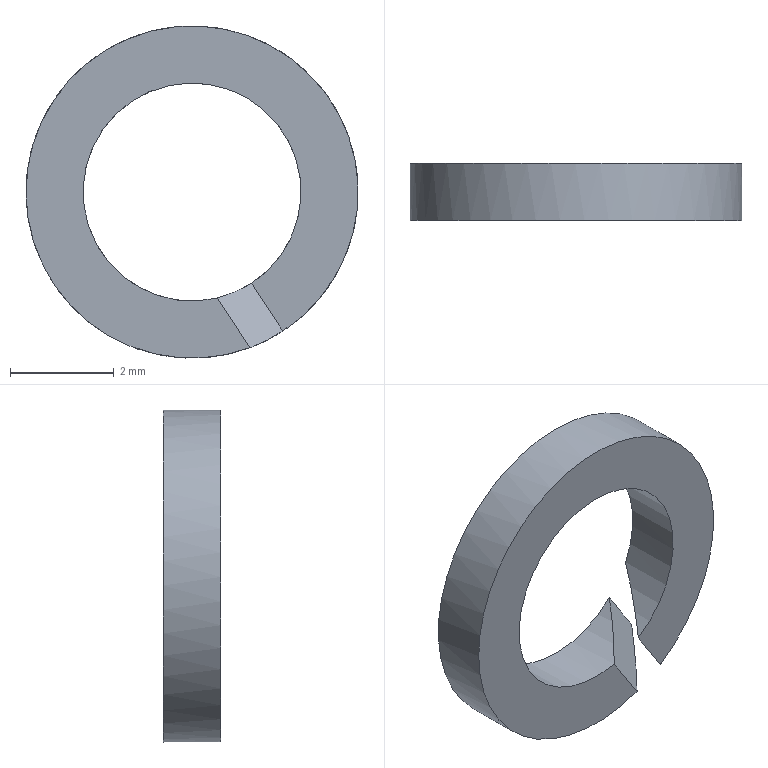Component | NX | SPRING_WASHER_4 | 1 solid | 6 faces | box 6.4 x 1.1 x 6.4 mm | volume 19 mm3 | plane 4 | cylinder 2 | commonest cylinder face diameters 6.4 x1 4.2 x1
STEP:
#1=CARTESIAN_POINT('',(0.,0.,0.));
#2=DIRECTION('',(0.,0.,1.));
#3=DIRECTION('',(1.,0.,0.));
#4=AXIS2_PLACEMENT_3D('',#1,#2,#3);
#5=CARTESIAN_POINT('',(21.566,-66.923,-95.444));
#6=VERTEX_POINT('',#5);
#7=CARTESIAN_POINT('',(22.064,-66.923,-94.914));
#8=VERTEX_POINT('',#7);
#9=CARTESIAN_POINT('',(19.5,-66.923,-93.));
#10=DIRECTION('',(0.,1.,0.));
#11=DIRECTION('',(0.5469,0.,-0.8372));
#12=AXIS2_PLACEMENT_3D('',#9,#10,#11);
#13=CIRCLE('',#12,3.2);
#14=CARTESIAN_POINT('',(19.5,-66.923,-93.));
#15=DIRECTION('',(0.,-1.,0.));
#16=DIRECTION('',(0.5469,0.,-0.8372));
#17=AXIS2_PLACEMENT_3D('',#14,#15,#16);
#18=CYLINDRICAL_SURFACE('',#17,3.2);
#19=CARTESIAN_POINT('',(12.566,0.));
#20=DIRECTION('',(-1.,0.));
#21=VECTOR('',#20,1.);
#22=LINE('',#19,#21);
#23=(GEOMETRIC_REPRESENTATION_CONTEXT(2)PARAMETRIC_REPRESENTATION_CONTEXT()REPRESENTATION_CONTEXT('',''));
#24=DEFINITIONAL_REPRESENTATION('',(#22),#23);
#25=PCURVE('',#18,#24);
#26=CARTESIAN_POINT('',(19.5,-66.923,-93.));
#27=DIRECTION('',(0.,-1.,0.));
#28=DIRECTION('',(0.5469,0.,-0.8372));
#29=AXIS2_PLACEMENT_3D('',#26,#27,#28);
#30=PLANE('',#29);
#31=CARTESIAN_POINT('',(3.2,-0.));
#32=CARTESIAN_POINT('',(3.2,-5.543));
#33=CARTESIAN_POINT('',(-1.6,-2.771));
#34=CARTESIAN_POINT('',(-6.4,0.));
#35=CARTESIAN_POINT('',(-1.6,2.771));
#36=CARTESIAN_POINT('',(3.2,5.543));
#37=CARTESIAN_POINT('',(3.2,-0.));
#38=(BOUNDED_CURVE()B_SPLINE_CURVE(2,(#31,#32,#33,#34,#35,#36,#37),.UNSPECIFIED.,.T.,.F.)B_SPLINE_CURVE_WITH_KNOTS((1,2,2,2,2,1),(-2.094,0.,2.094,4.189,6.283,8.378),.UNSPECIFIED.)CURVE()GEOMETRIC_REPRESENTATION_ITEM()RATIONAL_B_SPLINE_CURVE((1.,0.5,1.,0.5,1.,0.5,1.))REPRESENTATION_ITEM(''));
#39=(GEOMETRIC_REPRESENTATION_CONTEXT(2)PARAMETRIC_REPRESENTATION_CONTEXT()REPRESENTATION_CONTEXT('',''));
#40=DEFINITIONAL_REPRESENTATION('',(#38),#39);
#41=PCURVE('',#30,#40);
#42=SURFACE_CURVE('',#13,(#25,#41),.PCURVE_S1.);
#43=EDGE_CURVE('',#6,#8,#42,.T.);
#44=ORIENTED_EDGE('',*,*,#43,.F.);
#45=CARTESIAN_POINT('',(20.615,-68.023,-95.999));
#46=VERTEX_POINT('',#45);
#47=CARTESIAN_POINT('',(19.5,-67.316,-93.));
#48=DIRECTION('',(0.592,-0.7071,0.3867));
#49=DIRECTION('',(-0.592,-0.7071,-0.3867));
#50=AXIS2_PLACEMENT_3D('',#47,#48,#49);
#51=ELLIPSE('',#50,4.525,3.2);
#52=CARTESIAN_POINT('',(6.06,1.1));
#53=CARTESIAN_POINT('',(6.406,-0.));
#54=B_SPLINE_CURVE_WITH_KNOTS('',1,(#52,#53),.UNSPECIFIED.,.F.,.F.,(2,2),(1.348,1.694),.PIECEWISE_BEZIER_KNOTS.);
#55=(GEOMETRIC_REPRESENTATION_CONTEXT(2)PARAMETRIC_REPRESENTATION_CONTEXT()REPRESENTATION_CONTEXT('',''));
#56=DEFINITIONAL_REPRESENTATION('',(#54),#55);
#57=PCURVE('',#18,#56);
#58=CARTESIAN_POINT('',(23.341,-68.804,-101.6));
#59=DIRECTION('',(0.592,-0.7071,0.3867));
#60=DIRECTION('',(-0.592,-0.7071,-0.3867));
#61=AXIS2_PLACEMENT_3D('',#58,#59,#60);
#62=PLANE('',#61);
#63=CARTESIAN_POINT('',(-2.105,-9.3));
#64=DIRECTION('',(1.,-0.));
#65=AXIS2_PLACEMENT_2D('',#63,#64);
#66=ELLIPSE('',#65,4.525,3.2);
#67=(GEOMETRIC_REPRESENTATION_CONTEXT(2)PARAMETRIC_REPRESENTATION_CONTEXT()REPRESENTATION_CONTEXT('',''));
#68=DEFINITIONAL_REPRESENTATION('',(#66),#67);
#69=PCURVE('',#62,#68);
#70=SURFACE_CURVE('',#51,(#57,#69),.PCURVE_S1.);
#71=EDGE_CURVE('',#46,#6,#70,.T.);
#72=ORIENTED_EDGE('',*,*,#71,.F.);
#73=CARTESIAN_POINT('',(21.25,-68.023,-95.679));
#74=VERTEX_POINT('',#73);
#75=CARTESIAN_POINT('',(19.5,-68.023,-93.));
#76=DIRECTION('',(0.,1.,0.));
#77=DIRECTION('',(0.5469,0.,-0.8372));
#78=AXIS2_PLACEMENT_3D('',#75,#76,#77);
#79=CIRCLE('',#78,3.2);
#80=CARTESIAN_POINT('',(6.283,1.1));
#81=DIRECTION('',(-1.,0.));
#82=VECTOR('',#81,1.);
#83=LINE('',#80,#82);
#84=(GEOMETRIC_REPRESENTATION_CONTEXT(2)PARAMETRIC_REPRESENTATION_CONTEXT()REPRESENTATION_CONTEXT('',''));
#85=DEFINITIONAL_REPRESENTATION('',(#83),#84);
#86=PCURVE('',#18,#85);
#87=CARTESIAN_POINT('',(19.5,-68.023,-93.));
#88=DIRECTION('',(0.,-1.,0.));
#89=DIRECTION('',(0.5469,0.,-0.8372));
#90=AXIS2_PLACEMENT_3D('',#87,#88,#89);
#91=PLANE('',#90);
#92=CARTESIAN_POINT('',(3.2,-0.));
#93=CARTESIAN_POINT('',(3.2,-5.543));
#94=CARTESIAN_POINT('',(-1.6,-2.771));
#95=CARTESIAN_POINT('',(-6.4,0.));
#96=CARTESIAN_POINT('',(-1.6,2.771));
#97=CARTESIAN_POINT('',(3.2,5.543));
#98=CARTESIAN_POINT('',(3.2,-0.));
#99=(BOUNDED_CURVE()B_SPLINE_CURVE(2,(#92,#93,#94,#95,#96,#97,#98),.UNSPECIFIED.,.T.,.F.)B_SPLINE_CURVE_WITH_KNOTS((1,2,2,2,2,1),(-2.094,0.,2.094,4.189,6.283,8.378),.UNSPECIFIED.)CURVE()GEOMETRIC_REPRESENTATION_ITEM()RATIONAL_B_SPLINE_CURVE((1.,0.5,1.,0.5,1.,0.5,1.))REPRESENTATION_ITEM(''));
#100=(GEOMETRIC_REPRESENTATION_CONTEXT(2)PARAMETRIC_REPRESENTATION_CONTEXT()REPRESENTATION_CONTEXT('',''));
#101=DEFINITIONAL_REPRESENTATION('',(#99),#100);
#102=PCURVE('',#91,#101);
#103=SURFACE_CURVE('',#79,(#86,#102),.PCURVE_S1.);
#104=EDGE_CURVE('',#46,#74,#103,.T.);
#105=ORIENTED_EDGE('',*,*,#104,.T.);
#106=CARTESIAN_POINT('',(19.5,-68.023,-93.));
#107=DIRECTION('',(-0.592,0.7071,-0.3867));
#108=DIRECTION('',(-0.592,-0.7071,-0.3867));
#109=AXIS2_PLACEMENT_3D('',#106,#107,#108);
#110=ELLIPSE('',#109,4.525,3.2);
#111=CARTESIAN_POINT('',(0.3509,-0.));
#112=CARTESIAN_POINT('',(0.,1.1));
#113=B_SPLINE_CURVE_WITH_KNOTS('',1,(#111,#112),.UNSPECIFIED.,.F.,.F.,(2,2),(4.361,4.712),.PIECEWISE_BEZIER_KNOTS.);
#114=(GEOMETRIC_REPRESENTATION_CONTEXT(2)PARAMETRIC_REPRESENTATION_CONTEXT()REPRESENTATION_CONTEXT('',''));
#115=DEFINITIONAL_REPRESENTATION('',(#113),#114);
#116=PCURVE('',#18,#115);
#117=CARTESIAN_POINT('',(26.917,-65.239,-99.263));
#118=DIRECTION('',(-0.592,0.7071,-0.3867));
#119=DIRECTION('',(0.592,0.7071,0.3867));
#120=AXIS2_PLACEMENT_3D('',#117,#118,#119);
#121=PLANE('',#120);
#122=CARTESIAN_POINT('',(-3.936,-9.3));
#123=DIRECTION('',(-1.,-0.));
#124=AXIS2_PLACEMENT_2D('',#122,#123);
#125=ELLIPSE('',#124,4.525,3.2);
#126=(GEOMETRIC_REPRESENTATION_CONTEXT(2)PARAMETRIC_REPRESENTATION_CONTEXT()REPRESENTATION_CONTEXT('',''));
#127=DEFINITIONAL_REPRESENTATION('',(#125),#126);
#128=PCURVE('',#121,#127);
#129=SURFACE_CURVE('',#110,(#116,#128),.PCURVE_S1.);
#130=EDGE_CURVE('',#8,#74,#129,.T.);
#131=ORIENTED_EDGE('',*,*,#130,.F.);
#132=EDGE_LOOP('',(#44,#72,#105,#131));
#133=FACE_BOUND('',#132,.T.);
#134=ADVANCED_FACE('',(#133),#18,.T.);
#135=CARTESIAN_POINT('',(19.99,-68.023,-95.042));
#136=VERTEX_POINT('',#135);
#137=CARTESIAN_POINT('',(20.649,-68.023,-94.758));
#138=VERTEX_POINT('',#137);
#139=CARTESIAN_POINT('',(19.5,-68.023,-93.));
#140=DIRECTION('',(0.,1.,0.));
#141=DIRECTION('',(0.5469,0.,-0.8372));
#142=AXIS2_PLACEMENT_3D('',#139,#140,#141);
#143=CIRCLE('',#142,2.1);
#144=CARTESIAN_POINT('',(19.5,-66.923,-93.));
#145=DIRECTION('',(0.,-1.,0.));
#146=DIRECTION('',(0.5469,0.,-0.8372));
#147=AXIS2_PLACEMENT_3D('',#144,#145,#146);
#148=CYLINDRICAL_SURFACE('',#147,2.1);
#149=CARTESIAN_POINT('',(6.283,1.1));
#150=DIRECTION('',(-1.,0.));
#151=VECTOR('',#150,1.);
#152=LINE('',#149,#151);
#153=(GEOMETRIC_REPRESENTATION_CONTEXT(2)PARAMETRIC_REPRESENTATION_CONTEXT()REPRESENTATION_CONTEXT('',''));
#154=DEFINITIONAL_REPRESENTATION('',(#152),#153);
#155=PCURVE('',#148,#154);
#156=CARTESIAN_POINT('',(2.1,-0.));
#157=CARTESIAN_POINT('',(2.1,-3.637));
#158=CARTESIAN_POINT('',(-1.05,-1.819));
#159=CARTESIAN_POINT('',(-4.2,0.));
#160=CARTESIAN_POINT('',(-1.05,1.819));
#161=CARTESIAN_POINT('',(2.1,3.637));
#162=CARTESIAN_POINT('',(2.1,-0.));
#163=(BOUNDED_CURVE()B_SPLINE_CURVE(2,(#156,#157,#158,#159,#160,#161,#162),.UNSPECIFIED.,.T.,.F.)B_SPLINE_CURVE_WITH_KNOTS((1,2,2,2,2,1),(-2.094,0.,2.094,4.189,6.283,8.378),.UNSPECIFIED.)CURVE()GEOMETRIC_REPRESENTATION_ITEM()RATIONAL_B_SPLINE_CURVE((1.,0.5,1.,0.5,1.,0.5,1.))REPRESENTATION_ITEM(''));
#164=(GEOMETRIC_REPRESENTATION_CONTEXT(2)PARAMETRIC_REPRESENTATION_CONTEXT()REPRESENTATION_CONTEXT('',''));
#165=DEFINITIONAL_REPRESENTATION('',(#163),#164);
#166=PCURVE('',#91,#165);
#167=SURFACE_CURVE('',#143,(#155,#166),.PCURVE_S1.);
#168=EDGE_CURVE('',#136,#138,#167,.T.);
#169=ORIENTED_EDGE('',*,*,#168,.T.);
#170=CARTESIAN_POINT('',(21.399,-66.923,-93.896));
#171=VERTEX_POINT('',#170);
#172=CARTESIAN_POINT('',(19.5,-68.023,-93.));
#173=DIRECTION('',(-0.592,0.7071,-0.3867));
#174=DIRECTION('',(-0.592,-0.7071,-0.3867));
#175=AXIS2_PLACEMENT_3D('',#172,#173,#174);
#176=ELLIPSE('',#175,2.97,2.1);
#177=CARTESIAN_POINT('',(0.5513,0.));
#178=CARTESIAN_POINT('',(0.,1.1));
#179=B_SPLINE_CURVE_WITH_KNOTS('',1,(#177,#178),.UNSPECIFIED.,.F.,.F.,(2,2),(4.161,4.712),.PIECEWISE_BEZIER_KNOTS.);
#180=(GEOMETRIC_REPRESENTATION_CONTEXT(2)PARAMETRIC_REPRESENTATION_CONTEXT()REPRESENTATION_CONTEXT('',''));
#181=DEFINITIONAL_REPRESENTATION('',(#179),#180);
#182=PCURVE('',#148,#181);
#183=CARTESIAN_POINT('',(-3.936,-9.3));
#184=DIRECTION('',(-1.,-0.));
#185=AXIS2_PLACEMENT_2D('',#183,#184);
#186=ELLIPSE('',#185,2.97,2.1);
#187=(GEOMETRIC_REPRESENTATION_CONTEXT(2)PARAMETRIC_REPRESENTATION_CONTEXT()REPRESENTATION_CONTEXT('',''));
#188=DEFINITIONAL_REPRESENTATION('',(#186),#187);
#189=PCURVE('',#121,#188);
#190=SURFACE_CURVE('',#176,(#182,#189),.PCURVE_S1.);
#191=EDGE_CURVE('',#171,#138,#190,.T.);
#192=ORIENTED_EDGE('',*,*,#191,.F.);
#193=CARTESIAN_POINT('',(20.957,-66.923,-94.512));
#194=VERTEX_POINT('',#193);
#195=CARTESIAN_POINT('',(19.5,-66.923,-93.));
#196=DIRECTION('',(0.,1.,0.));
#197=DIRECTION('',(0.5469,0.,-0.8372));
#198=AXIS2_PLACEMENT_3D('',#195,#196,#197);
#199=CIRCLE('',#198,2.1);
#200=CARTESIAN_POINT('',(12.566,0.));
#201=DIRECTION('',(-1.,0.));
#202=VECTOR('',#201,1.);
#203=LINE('',#200,#202);
#204=(GEOMETRIC_REPRESENTATION_CONTEXT(2)PARAMETRIC_REPRESENTATION_CONTEXT()REPRESENTATION_CONTEXT('',''));
#205=DEFINITIONAL_REPRESENTATION('',(#203),#204);
#206=PCURVE('',#148,#205);
#207=CARTESIAN_POINT('',(2.1,-0.));
#208=CARTESIAN_POINT('',(2.1,-3.637));
#209=CARTESIAN_POINT('',(-1.05,-1.819));
#210=CARTESIAN_POINT('',(-4.2,0.));
#211=CARTESIAN_POINT('',(-1.05,1.819));
#212=CARTESIAN_POINT('',(2.1,3.637));
#213=CARTESIAN_POINT('',(2.1,-0.));
#214=(BOUNDED_CURVE()B_SPLINE_CURVE(2,(#207,#208,#209,#210,#211,#212,#213),.UNSPECIFIED.,.T.,.F.)B_SPLINE_CURVE_WITH_KNOTS((1,2,2,2,2,1),(-2.094,0.,2.094,4.189,6.283,8.378),.UNSPECIFIED.)CURVE()GEOMETRIC_REPRESENTATION_ITEM()RATIONAL_B_SPLINE_CURVE((1.,0.5,1.,0.5,1.,0.5,1.))REPRESENTATION_ITEM(''));
#215=(GEOMETRIC_REPRESENTATION_CONTEXT(2)PARAMETRIC_REPRESENTATION_CONTEXT()REPRESENTATION_CONTEXT('',''));
#216=DEFINITIONAL_REPRESENTATION('',(#214),#215);
#217=PCURVE('',#30,#216);
#218=SURFACE_CURVE('',#199,(#206,#217),.PCURVE_S1.);
#219=EDGE_CURVE('',#194,#171,#218,.T.);
#220=ORIENTED_EDGE('',*,*,#219,.F.);
#221=CARTESIAN_POINT('',(19.5,-67.316,-93.));
#222=DIRECTION('',(0.592,-0.7071,0.3867));
#223=DIRECTION('',(-0.592,-0.7071,-0.3867));
#224=AXIS2_PLACEMENT_3D('',#221,#222,#223);
#225=ELLIPSE('',#224,2.97,2.1);
#226=CARTESIAN_POINT('',(5.94,1.1));
#227=CARTESIAN_POINT('',(6.471,-0.));
#228=B_SPLINE_CURVE_WITH_KNOTS('',1,(#226,#227),.UNSPECIFIED.,.F.,.F.,(2,2),(1.227,1.759),.PIECEWISE_BEZIER_KNOTS.);
#229=(GEOMETRIC_REPRESENTATION_CONTEXT(2)PARAMETRIC_REPRESENTATION_CONTEXT()REPRESENTATION_CONTEXT('',''));
#230=DEFINITIONAL_REPRESENTATION('',(#228),#229);
#231=PCURVE('',#148,#230);
#232=CARTESIAN_POINT('',(-2.105,-9.3));
#233=DIRECTION('',(1.,-0.));
#234=AXIS2_PLACEMENT_2D('',#232,#233);
#235=ELLIPSE('',#234,2.97,2.1);
#236=(GEOMETRIC_REPRESENTATION_CONTEXT(2)PARAMETRIC_REPRESENTATION_CONTEXT()REPRESENTATION_CONTEXT('',''));
#237=DEFINITIONAL_REPRESENTATION('',(#235),#236);
#238=PCURVE('',#62,#237);
#239=SURFACE_CURVE('',#225,(#231,#238),.PCURVE_S1.);
#240=EDGE_CURVE('',#136,#194,#239,.T.);
#241=ORIENTED_EDGE('',*,*,#240,.F.);
#242=EDGE_LOOP('',(#169,#192,#220,#241));
#243=FACE_BOUND('',#242,.F.);
#244=ADVANCED_FACE('',(#243),#148,.F.);
#245=CARTESIAN_POINT('',(19.829,-66.923,-92.785));
#246=DIRECTION('',(-0.5469,0.,0.8372));
#247=VECTOR('',#246,1.);
#248=LINE('',#245,#247);
#249=CARTESIAN_POINT('',(-0.,0.3929));
#250=DIRECTION('',(-1.,0.));
#251=VECTOR('',#250,1.);
#252=LINE('',#249,#251);
#253=(GEOMETRIC_REPRESENTATION_CONTEXT(2)PARAMETRIC_REPRESENTATION_CONTEXT()REPRESENTATION_CONTEXT('',''));
#254=DEFINITIONAL_REPRESENTATION('',(#252),#253);
#255=PCURVE('',#30,#254);
#256=CARTESIAN_POINT('',(-2.66,-9.3));
#257=DIRECTION('',(0.,-1.));
#258=VECTOR('',#257,1.);
#259=LINE('',#256,#258);
#260=(GEOMETRIC_REPRESENTATION_CONTEXT(2)PARAMETRIC_REPRESENTATION_CONTEXT()REPRESENTATION_CONTEXT('',''));
#261=DEFINITIONAL_REPRESENTATION('',(#259),#260);
#262=PCURVE('',#62,#261);
#263=SURFACE_CURVE('',#248,(#255,#262),.PCURVE_S1.);
#264=EDGE_CURVE('',#6,#194,#263,.T.);
#265=ORIENTED_EDGE('',*,*,#264,.F.);
#266=ORIENTED_EDGE('',*,*,#43,.T.);
#267=CARTESIAN_POINT('',(20.421,-66.923,-92.398));
#268=DIRECTION('',(0.5469,0.,-0.8372));
#269=VECTOR('',#268,1.);
#270=LINE('',#267,#269);
#271=CARTESIAN_POINT('',(0.,1.1));
#272=DIRECTION('',(1.,0.));
#273=VECTOR('',#272,1.);
#274=LINE('',#271,#273);
#275=(GEOMETRIC_REPRESENTATION_CONTEXT(2)PARAMETRIC_REPRESENTATION_CONTEXT()REPRESENTATION_CONTEXT('',''));
#276=DEFINITIONAL_REPRESENTATION('',(#274),#275);
#277=PCURVE('',#30,#276);
#278=CARTESIAN_POINT('',(-2.38,-9.3));
#279=DIRECTION('',(0.,1.));
#280=VECTOR('',#279,1.);
#281=LINE('',#278,#280);
#282=(GEOMETRIC_REPRESENTATION_CONTEXT(2)PARAMETRIC_REPRESENTATION_CONTEXT()REPRESENTATION_CONTEXT('',''));
#283=DEFINITIONAL_REPRESENTATION('',(#281),#282);
#284=PCURVE('',#121,#283);
#285=SURFACE_CURVE('',#270,(#277,#284),.PCURVE_S1.);
#286=EDGE_CURVE('',#171,#8,#285,.T.);
#287=ORIENTED_EDGE('',*,*,#286,.F.);
#288=ORIENTED_EDGE('',*,*,#219,.F.);
#289=EDGE_LOOP('',(#265,#266,#287,#288));
#290=FACE_BOUND('',#289,.T.);
#291=ADVANCED_FACE('',(#290),#30,.F.);
#292=ORIENTED_EDGE('',*,*,#104,.F.);
#293=CARTESIAN_POINT('',(18.908,-68.023,-93.387));
#294=DIRECTION('',(-0.5469,0.,0.8372));
#295=VECTOR('',#294,1.);
#296=LINE('',#293,#295);
#297=CARTESIAN_POINT('',(0.,-0.7071));
#298=DIRECTION('',(-1.,0.));
#299=VECTOR('',#298,1.);
#300=LINE('',#297,#299);
#301=(GEOMETRIC_REPRESENTATION_CONTEXT(2)PARAMETRIC_REPRESENTATION_CONTEXT()REPRESENTATION_CONTEXT('',''));
#302=DEFINITIONAL_REPRESENTATION('',(#300),#301);
#303=PCURVE('',#91,#302);
#304=CARTESIAN_POINT('',(-1.105,-9.3));
#305=DIRECTION('',(0.,-1.));
#306=VECTOR('',#305,1.);
#307=LINE('',#304,#306);
#308=(GEOMETRIC_REPRESENTATION_CONTEXT(2)PARAMETRIC_REPRESENTATION_CONTEXT()REPRESENTATION_CONTEXT('',''));
#309=DEFINITIONAL_REPRESENTATION('',(#307),#308);
#310=PCURVE('',#62,#309);
#311=SURFACE_CURVE('',#296,(#303,#310),.PCURVE_S1.);
#312=EDGE_CURVE('',#46,#136,#311,.T.);
#313=ORIENTED_EDGE('',*,*,#312,.T.);
#314=ORIENTED_EDGE('',*,*,#168,.T.);
#315=CARTESIAN_POINT('',(19.5,-68.023,-93.));
#316=DIRECTION('',(0.5469,0.,-0.8372));
#317=VECTOR('',#316,1.);
#318=LINE('',#315,#317);
#319=CARTESIAN_POINT('',(0.,0.));
#320=DIRECTION('',(1.,0.));
#321=VECTOR('',#320,1.);
#322=LINE('',#319,#321);
#323=(GEOMETRIC_REPRESENTATION_CONTEXT(2)PARAMETRIC_REPRESENTATION_CONTEXT()REPRESENTATION_CONTEXT('',''));
#324=DEFINITIONAL_REPRESENTATION('',(#322),#323);
#325=PCURVE('',#91,#324);
#326=CARTESIAN_POINT('',(-3.936,-9.3));
#327=DIRECTION('',(0.,1.));
#328=VECTOR('',#327,1.);
#329=LINE('',#326,#328);
#330=(GEOMETRIC_REPRESENTATION_CONTEXT(2)PARAMETRIC_REPRESENTATION_CONTEXT()REPRESENTATION_CONTEXT('',''));
#331=DEFINITIONAL_REPRESENTATION('',(#329),#330);
#332=PCURVE('',#121,#331);
#333=SURFACE_CURVE('',#318,(#325,#332),.PCURVE_S1.);
#334=EDGE_CURVE('',#138,#74,#333,.T.);
#335=ORIENTED_EDGE('',*,*,#334,.T.);
#336=EDGE_LOOP('',(#292,#313,#314,#335));
#337=FACE_BOUND('',#336,.T.);
#338=ADVANCED_FACE('',(#337),#91,.T.);
#339=ORIENTED_EDGE('',*,*,#286,.T.);
#340=ORIENTED_EDGE('',*,*,#130,.T.);
#341=ORIENTED_EDGE('',*,*,#334,.F.);
#342=ORIENTED_EDGE('',*,*,#191,.F.);
#343=EDGE_LOOP('',(#339,#340,#341,#342));
#344=FACE_BOUND('',#343,.T.);
#345=ADVANCED_FACE('',(#344),#121,.T.);
#346=ORIENTED_EDGE('',*,*,#264,.T.);
#347=ORIENTED_EDGE('',*,*,#240,.F.);
#348=ORIENTED_EDGE('',*,*,#312,.F.);
#349=ORIENTED_EDGE('',*,*,#71,.T.);
#350=EDGE_LOOP('',(#346,#347,#348,#349));
#351=FACE_BOUND('',#350,.T.);
#352=ADVANCED_FACE('',(#351),#62,.T.);
#353=CLOSED_SHELL('',(#134,#244,#291,#338,#345,#352));
#354=MANIFOLD_SOLID_BREP('',#353);
#355=(LENGTH_UNIT()NAMED_UNIT(*)SI_UNIT(.MILLI.,.METRE.));
#356=UNCERTAINTY_MEASURE_WITH_UNIT(LENGTH_MEASURE(0.01),#355,'','');
#357=(NAMED_UNIT(*)PLANE_ANGLE_UNIT()SI_UNIT($,.RADIAN.));
#358=(NAMED_UNIT(*)SI_UNIT($,.STERADIAN.)SOLID_ANGLE_UNIT());
#359=(GEOMETRIC_REPRESENTATION_CONTEXT(3)GLOBAL_UNCERTAINTY_ASSIGNED_CONTEXT((#356))GLOBAL_UNIT_ASSIGNED_CONTEXT((#355,#357,#358))REPRESENTATION_CONTEXT('',''));
#360=ADVANCED_BREP_SHAPE_REPRESENTATION('',(#4,#354),#359);